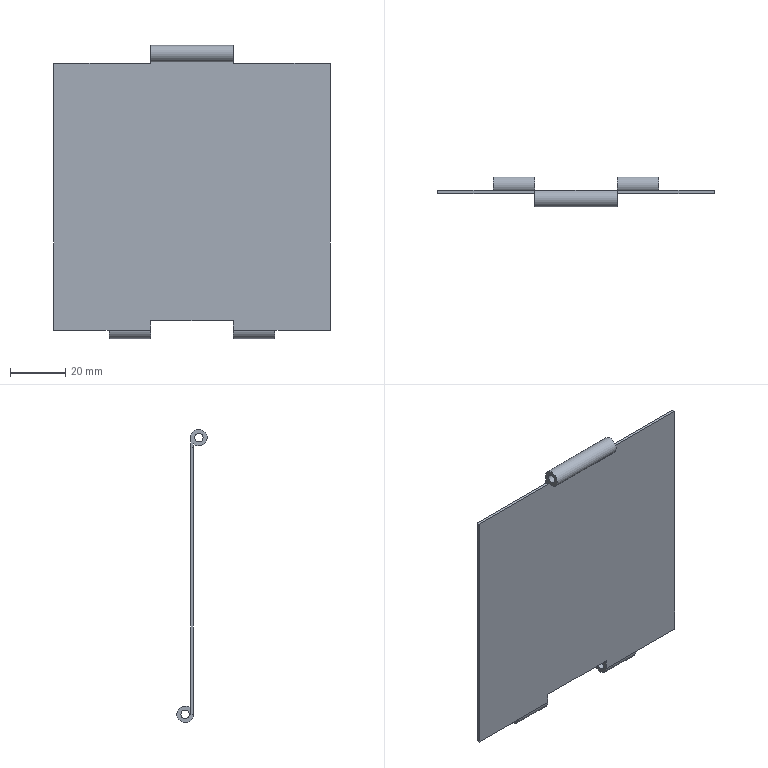Component | NX | PART_3_2 | 1 solid | 21 faces | volume 10829 mm3 | plane 15 | cylinder 6 | commonest cylinder face diameters 6 x3 3 x3